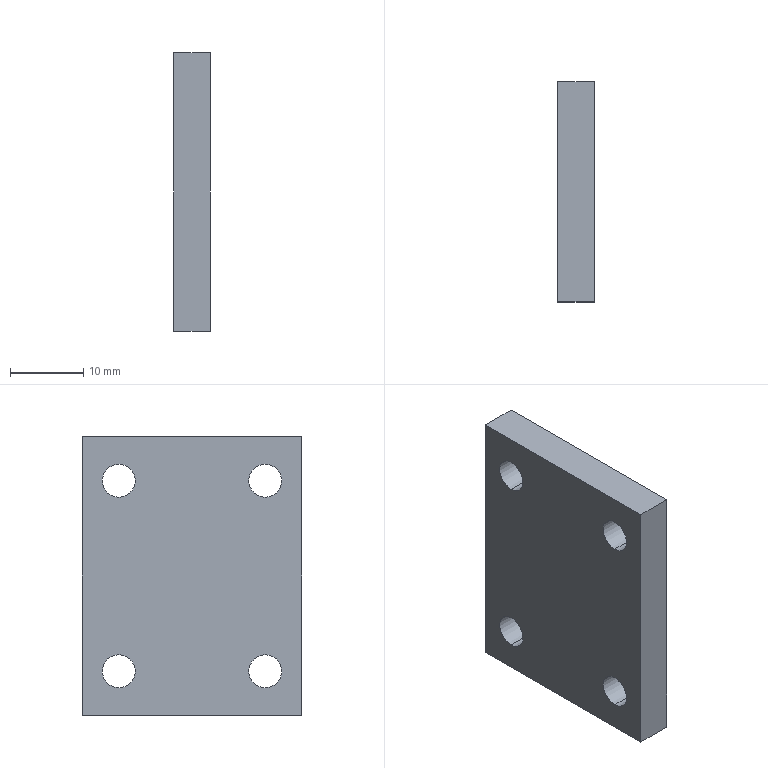Component | SolidWorks | DC-024-30-1 | 1 solid | 14 faces | box 5 x 30 x 38 mm | volume 5382 mm3 | cylinder 8 | plane 6 | commonest cylinder face diameters 4.5 x8
build123d program:
from build123d import *

# Parameters (mm, degrees)
SKETCH1_W                  = 38
SKETCH1_H                  = 30
BOSS_EXTRUDE1_DEPTH        = 2.5
F_4_5_4_5_DIAMETER_HOLE1_D = 4.5


with BuildPart() as part:
    # Sketch1 → Boss-Extrude1 (new, symmetric)
    with BuildSketch(Plane.XY):
        Rectangle(SKETCH1_W, SKETCH1_H)
    extrude(amount=BOSS_EXTRUDE1_DEPTH, both=True)

    # 4.5 _4.5_ Diameter Hole1 (through all)
    with Locations(Plane.XY.offset(2.5)):
        with Locations((-13, 10), (-13, -10), (13, -10), (13, 10)):
            Hole(F_4_5_4_5_DIAMETER_HOLE1_D / 2)


solid = part.part

# Placed as in the assembly
solid = solid.moved(Location((-65.833, 220.806, 37), (0, 90, 0)))
STEP:
#1=COLOUR_RGB('',0.7922,0.8196,0.9333);
#2=FILL_AREA_STYLE_COLOUR('',#1);
#3=FILL_AREA_STYLE('',(#2));
#4=SURFACE_STYLE_FILL_AREA(#3);
#5=SURFACE_SIDE_STYLE('',(#4));
#6=SURFACE_STYLE_USAGE(.BOTH.,#5);
#7=PRESENTATION_STYLE_ASSIGNMENT((#6));
#8=CARTESIAN_POINT('',(-2.69,9.087,2.057));
#9=VERTEX_POINT('',#8);
#10=CARTESIAN_POINT('',(-2.69,9.087,1.88));
#11=VERTEX_POINT('',#10);
#12=CARTESIAN_POINT('',(-2.69,9.087,1.969));
#13=DIRECTION('',(1.,-0.,0.));
#14=DIRECTION('',(0.,0.,-1.));
#15=AXIS2_PLACEMENT_3D('',#12,#13,#14);
#16=CIRCLE('',#15,0.08858);
#17=EDGE_CURVE('',#9,#11,#16,.T.);
#18=ORIENTED_EDGE('',*,*,#17,.F.);
#19=CARTESIAN_POINT('',(-2.493,9.087,2.057));
#20=VERTEX_POINT('',#19);
#21=CARTESIAN_POINT('',(-2.493,9.087,2.057));
#22=DIRECTION('',(1.,-0.,0.));
#23=VECTOR('',#22,39.37);
#24=LINE('',#21,#23);
#25=EDGE_CURVE('',#9,#20,#24,.T.);
#26=ORIENTED_EDGE('',*,*,#25,.T.);
#27=CARTESIAN_POINT('',(-2.493,9.087,1.88));
#28=VERTEX_POINT('',#27);
#29=CARTESIAN_POINT('',(-2.493,9.087,1.969));
#30=DIRECTION('',(1.,-0.,0.));
#31=DIRECTION('',(0.,0.,-1.));
#32=AXIS2_PLACEMENT_3D('',#29,#30,#31);
#33=CIRCLE('',#32,0.08858);
#34=EDGE_CURVE('',#20,#28,#33,.T.);
#35=ORIENTED_EDGE('',*,*,#34,.T.);
#36=CARTESIAN_POINT('',(-2.493,9.087,1.88));
#37=DIRECTION('',(1.,-0.,0.));
#38=VECTOR('',#37,39.37);
#39=LINE('',#36,#38);
#40=EDGE_CURVE('',#11,#28,#39,.T.);
#41=ORIENTED_EDGE('',*,*,#40,.F.);
#42=EDGE_LOOP('',(#18,#26,#35,#41));
#43=FACE_OUTER_BOUND('',#42,.T.);
#44=CARTESIAN_POINT('',(-2.493,9.087,1.969));
#45=DIRECTION('',(1.,-0.,0.));
#46=DIRECTION('',(0.,0.,-1.));
#47=AXIS2_PLACEMENT_3D('',#44,#45,#46);
#48=CYLINDRICAL_SURFACE('',#47,0.08858);
#49=ADVANCED_FACE('',(#43),#48,.F.);
#50=CARTESIAN_POINT('',(-2.69,8.299,2.057));
#51=VERTEX_POINT('',#50);
#52=CARTESIAN_POINT('',(-2.69,8.299,1.88));
#53=VERTEX_POINT('',#52);
#54=CARTESIAN_POINT('',(-2.69,8.299,1.969));
#55=DIRECTION('',(1.,-0.,0.));
#56=DIRECTION('',(0.,0.,-1.));
#57=AXIS2_PLACEMENT_3D('',#54,#55,#56);
#58=CIRCLE('',#57,0.08858);
#59=EDGE_CURVE('',#51,#53,#58,.T.);
#60=ORIENTED_EDGE('',*,*,#59,.F.);
#61=CARTESIAN_POINT('',(-2.493,8.299,2.057));
#62=VERTEX_POINT('',#61);
#63=CARTESIAN_POINT('',(-2.493,8.299,2.057));
#64=DIRECTION('',(1.,-0.,0.));
#65=VECTOR('',#64,39.37);
#66=LINE('',#63,#65);
#67=EDGE_CURVE('',#51,#62,#66,.T.);
#68=ORIENTED_EDGE('',*,*,#67,.T.);
#69=CARTESIAN_POINT('',(-2.493,8.299,1.88));
#70=VERTEX_POINT('',#69);
#71=CARTESIAN_POINT('',(-2.493,8.299,1.969));
#72=DIRECTION('',(1.,-0.,0.));
#73=DIRECTION('',(0.,0.,-1.));
#74=AXIS2_PLACEMENT_3D('',#71,#72,#73);
#75=CIRCLE('',#74,0.08858);
#76=EDGE_CURVE('',#62,#70,#75,.T.);
#77=ORIENTED_EDGE('',*,*,#76,.T.);
#78=CARTESIAN_POINT('',(-2.493,8.299,1.88));
#79=DIRECTION('',(1.,-0.,0.));
#80=VECTOR('',#79,39.37);
#81=LINE('',#78,#80);
#82=EDGE_CURVE('',#53,#70,#81,.T.);
#83=ORIENTED_EDGE('',*,*,#82,.F.);
#84=EDGE_LOOP('',(#60,#68,#77,#83));
#85=FACE_OUTER_BOUND('',#84,.T.);
#86=CARTESIAN_POINT('',(-2.493,8.299,1.969));
#87=DIRECTION('',(1.,-0.,0.));
#88=DIRECTION('',(0.,0.,-1.));
#89=AXIS2_PLACEMENT_3D('',#86,#87,#88);
#90=CYLINDRICAL_SURFACE('',#89,0.08858);
#91=ADVANCED_FACE('',(#85),#90,.F.);
#92=CARTESIAN_POINT('',(-2.69,8.299,1.033));
#93=VERTEX_POINT('',#92);
#94=CARTESIAN_POINT('',(-2.69,8.299,0.8563));
#95=VERTEX_POINT('',#94);
#96=CARTESIAN_POINT('',(-2.69,8.299,0.9449));
#97=DIRECTION('',(1.,-0.,0.));
#98=DIRECTION('',(0.,0.,-1.));
#99=AXIS2_PLACEMENT_3D('',#96,#97,#98);
#100=CIRCLE('',#99,0.08858);
#101=EDGE_CURVE('',#93,#95,#100,.T.);
#102=ORIENTED_EDGE('',*,*,#101,.F.);
#103=CARTESIAN_POINT('',(-2.493,8.299,1.033));
#104=VERTEX_POINT('',#103);
#105=CARTESIAN_POINT('',(-2.493,8.299,1.033));
#106=DIRECTION('',(1.,-0.,0.));
#107=VECTOR('',#106,39.37);
#108=LINE('',#105,#107);
#109=EDGE_CURVE('',#93,#104,#108,.T.);
#110=ORIENTED_EDGE('',*,*,#109,.T.);
#111=CARTESIAN_POINT('',(-2.493,8.299,0.8563));
#112=VERTEX_POINT('',#111);
#113=CARTESIAN_POINT('',(-2.493,8.299,0.9449));
#114=DIRECTION('',(1.,-0.,0.));
#115=DIRECTION('',(0.,0.,-1.));
#116=AXIS2_PLACEMENT_3D('',#113,#114,#115);
#117=CIRCLE('',#116,0.08858);
#118=EDGE_CURVE('',#104,#112,#117,.T.);
#119=ORIENTED_EDGE('',*,*,#118,.T.);
#120=CARTESIAN_POINT('',(-2.493,8.299,0.8563));
#121=DIRECTION('',(1.,-0.,0.));
#122=VECTOR('',#121,39.37);
#123=LINE('',#120,#122);
#124=EDGE_CURVE('',#95,#112,#123,.T.);
#125=ORIENTED_EDGE('',*,*,#124,.F.);
#126=EDGE_LOOP('',(#102,#110,#119,#125));
#127=FACE_OUTER_BOUND('',#126,.T.);
#128=CARTESIAN_POINT('',(-2.493,8.299,0.9449));
#129=DIRECTION('',(1.,-0.,0.));
#130=DIRECTION('',(0.,0.,-1.));
#131=AXIS2_PLACEMENT_3D('',#128,#129,#130);
#132=CYLINDRICAL_SURFACE('',#131,0.08858);
#133=ADVANCED_FACE('',(#127),#132,.F.);
#134=CARTESIAN_POINT('',(-2.69,9.087,1.033));
#135=VERTEX_POINT('',#134);
#136=CARTESIAN_POINT('',(-2.69,9.087,0.8563));
#137=VERTEX_POINT('',#136);
#138=CARTESIAN_POINT('',(-2.69,9.087,0.9449));
#139=DIRECTION('',(1.,-0.,0.));
#140=DIRECTION('',(0.,0.,-1.));
#141=AXIS2_PLACEMENT_3D('',#138,#139,#140);
#142=CIRCLE('',#141,0.08858);
#143=EDGE_CURVE('',#135,#137,#142,.T.);
#144=ORIENTED_EDGE('',*,*,#143,.F.);
#145=CARTESIAN_POINT('',(-2.493,9.087,1.033));
#146=VERTEX_POINT('',#145);
#147=CARTESIAN_POINT('',(-2.493,9.087,1.033));
#148=DIRECTION('',(1.,-0.,0.));
#149=VECTOR('',#148,39.37);
#150=LINE('',#147,#149);
#151=EDGE_CURVE('',#135,#146,#150,.T.);
#152=ORIENTED_EDGE('',*,*,#151,.T.);
#153=CARTESIAN_POINT('',(-2.493,9.087,0.8563));
#154=VERTEX_POINT('',#153);
#155=CARTESIAN_POINT('',(-2.493,9.087,0.9449));
#156=DIRECTION('',(1.,-0.,0.));
#157=DIRECTION('',(0.,0.,-1.));
#158=AXIS2_PLACEMENT_3D('',#155,#156,#157);
#159=CIRCLE('',#158,0.08858);
#160=EDGE_CURVE('',#146,#154,#159,.T.);
#161=ORIENTED_EDGE('',*,*,#160,.T.);
#162=CARTESIAN_POINT('',(-2.493,9.087,0.8563));
#163=DIRECTION('',(1.,-0.,0.));
#164=VECTOR('',#163,39.37);
#165=LINE('',#162,#164);
#166=EDGE_CURVE('',#137,#154,#165,.T.);
#167=ORIENTED_EDGE('',*,*,#166,.F.);
#168=EDGE_LOOP('',(#144,#152,#161,#167));
#169=FACE_OUTER_BOUND('',#168,.T.);
#170=CARTESIAN_POINT('',(-2.493,9.087,0.9449));
#171=DIRECTION('',(1.,-0.,0.));
#172=DIRECTION('',(0.,0.,-1.));
#173=AXIS2_PLACEMENT_3D('',#170,#171,#172);
#174=CYLINDRICAL_SURFACE('',#173,0.08858);
#175=ADVANCED_FACE('',(#169),#174,.F.);
#176=CARTESIAN_POINT('',(-2.69,9.284,2.205));
#177=VERTEX_POINT('',#176);
#178=CARTESIAN_POINT('',(-2.69,8.103,2.205));
#179=VERTEX_POINT('',#178);
#180=CARTESIAN_POINT('',(-2.69,8.103,2.205));
#181=DIRECTION('',(-0.,-1.,-0.));
#182=VECTOR('',#181,39.37);
#183=LINE('',#180,#182);
#184=EDGE_CURVE('',#177,#179,#183,.T.);
#185=ORIENTED_EDGE('',*,*,#184,.T.);
#186=CARTESIAN_POINT('',(-2.493,8.103,2.205));
#187=VERTEX_POINT('',#186);
#188=CARTESIAN_POINT('',(-2.493,8.103,2.205));
#189=DIRECTION('',(-1.,0.,-0.));
#190=VECTOR('',#189,39.37);
#191=LINE('',#188,#190);
#192=EDGE_CURVE('',#187,#179,#191,.T.);
#193=ORIENTED_EDGE('',*,*,#192,.F.);
#194=CARTESIAN_POINT('',(-2.493,9.284,2.205));
#195=VERTEX_POINT('',#194);
#196=CARTESIAN_POINT('',(-2.493,8.103,2.205));
#197=DIRECTION('',(-0.,-1.,-0.));
#198=VECTOR('',#197,39.37);
#199=LINE('',#196,#198);
#200=EDGE_CURVE('',#195,#187,#199,.T.);
#201=ORIENTED_EDGE('',*,*,#200,.F.);
#202=CARTESIAN_POINT('',(-2.493,9.284,2.205));
#203=DIRECTION('',(-1.,0.,-0.));
#204=VECTOR('',#203,39.37);
#205=LINE('',#202,#204);
#206=EDGE_CURVE('',#195,#177,#205,.T.);
#207=ORIENTED_EDGE('',*,*,#206,.T.);
#208=EDGE_LOOP('',(#185,#193,#201,#207));
#209=FACE_OUTER_BOUND('',#208,.T.);
#210=CARTESIAN_POINT('',(-2.493,8.103,2.205));
#211=DIRECTION('',(0.,0.,-1.));
#212=DIRECTION('',(-1.,0.,-0.));
#213=AXIS2_PLACEMENT_3D('',#210,#211,#212);
#214=PLANE('',#213);
#215=ADVANCED_FACE('',(#209),#214,.F.);
#216=CARTESIAN_POINT('',(-2.69,8.103,0.7087));
#217=VERTEX_POINT('',#216);
#218=CARTESIAN_POINT('',(-2.69,8.103,0.7087));
#219=DIRECTION('',(0.,0.,-1.));
#220=VECTOR('',#219,39.37);
#221=LINE('',#218,#220);
#222=EDGE_CURVE('',#179,#217,#221,.T.);
#223=ORIENTED_EDGE('',*,*,#222,.T.);
#224=CARTESIAN_POINT('',(-2.493,8.103,0.7087));
#225=VERTEX_POINT('',#224);
#226=CARTESIAN_POINT('',(-2.493,8.103,0.7087));
#227=DIRECTION('',(-1.,0.,-0.));
#228=VECTOR('',#227,39.37);
#229=LINE('',#226,#228);
#230=EDGE_CURVE('',#225,#217,#229,.T.);
#231=ORIENTED_EDGE('',*,*,#230,.F.);
#232=CARTESIAN_POINT('',(-2.493,8.103,0.7087));
#233=DIRECTION('',(0.,0.,-1.));
#234=VECTOR('',#233,39.37);
#235=LINE('',#232,#234);
#236=EDGE_CURVE('',#187,#225,#235,.T.);
#237=ORIENTED_EDGE('',*,*,#236,.F.);
#238=ORIENTED_EDGE('',*,*,#192,.T.);
#239=EDGE_LOOP('',(#223,#231,#237,#238));
#240=FACE_OUTER_BOUND('',#239,.T.);
#241=CARTESIAN_POINT('',(-2.493,8.103,0.7087));
#242=DIRECTION('',(0.,1.,0.));
#243=DIRECTION('',(-0.,-0.,1.));
#244=AXIS2_PLACEMENT_3D('',#241,#242,#243);
#245=PLANE('',#244);
#246=ADVANCED_FACE('',(#240),#245,.F.);
#247=CARTESIAN_POINT('',(-2.69,9.284,0.7087));
#248=VERTEX_POINT('',#247);
#249=CARTESIAN_POINT('',(-2.69,8.103,0.7087));
#250=DIRECTION('',(0.,1.,0.));
#251=VECTOR('',#250,39.37);
#252=LINE('',#249,#251);
#253=EDGE_CURVE('',#217,#248,#252,.T.);
#254=ORIENTED_EDGE('',*,*,#253,.T.);
#255=CARTESIAN_POINT('',(-2.493,9.284,0.7087));
#256=VERTEX_POINT('',#255);
#257=CARTESIAN_POINT('',(-2.493,9.284,0.7087));
#258=DIRECTION('',(-1.,0.,-0.));
#259=VECTOR('',#258,39.37);
#260=LINE('',#257,#259);
#261=EDGE_CURVE('',#256,#248,#260,.T.);
#262=ORIENTED_EDGE('',*,*,#261,.F.);
#263=CARTESIAN_POINT('',(-2.493,8.103,0.7087));
#264=DIRECTION('',(0.,1.,0.));
#265=VECTOR('',#264,39.37);
#266=LINE('',#263,#265);
#267=EDGE_CURVE('',#225,#256,#266,.T.);
#268=ORIENTED_EDGE('',*,*,#267,.F.);
#269=ORIENTED_EDGE('',*,*,#230,.T.);
#270=EDGE_LOOP('',(#254,#262,#268,#269));
#271=FACE_OUTER_BOUND('',#270,.T.);
#272=CARTESIAN_POINT('',(-2.493,8.103,0.7087));
#273=DIRECTION('',(-0.,-0.,1.));
#274=DIRECTION('',(1.,-0.,0.));
#275=AXIS2_PLACEMENT_3D('',#272,#273,#274);
#276=PLANE('',#275);
#277=ADVANCED_FACE('',(#271),#276,.F.);
#278=CARTESIAN_POINT('',(-2.69,9.284,0.7087));
#279=DIRECTION('',(-0.,-0.,1.));
#280=VECTOR('',#279,39.37);
#281=LINE('',#278,#280);
#282=EDGE_CURVE('',#248,#177,#281,.T.);
#283=ORIENTED_EDGE('',*,*,#282,.T.);
#284=ORIENTED_EDGE('',*,*,#206,.F.);
#285=CARTESIAN_POINT('',(-2.493,9.284,0.7087));
#286=DIRECTION('',(-0.,-0.,1.));
#287=VECTOR('',#286,39.37);
#288=LINE('',#285,#287);
#289=EDGE_CURVE('',#256,#195,#288,.T.);
#290=ORIENTED_EDGE('',*,*,#289,.F.);
#291=ORIENTED_EDGE('',*,*,#261,.T.);
#292=EDGE_LOOP('',(#283,#284,#290,#291));
#293=FACE_OUTER_BOUND('',#292,.T.);
#294=CARTESIAN_POINT('',(-2.493,9.284,0.7087));
#295=DIRECTION('',(-0.,-1.,-0.));
#296=DIRECTION('',(0.,0.,-1.));
#297=AXIS2_PLACEMENT_3D('',#294,#295,#296);
#298=PLANE('',#297);
#299=ADVANCED_FACE('',(#293),#298,.F.);
#300=CARTESIAN_POINT('',(-2.493,9.087,1.969));
#301=DIRECTION('',(1.,-0.,0.));
#302=DIRECTION('',(0.,0.,-1.));
#303=AXIS2_PLACEMENT_3D('',#300,#301,#302);
#304=CIRCLE('',#303,0.08858);
#305=EDGE_CURVE('',#28,#20,#304,.T.);
#306=ORIENTED_EDGE('',*,*,#305,.F.);
#307=ORIENTED_EDGE('',*,*,#34,.F.);
#308=EDGE_LOOP('',(#306,#307));
#309=FACE_BOUND('',#308,.T.);
#310=CARTESIAN_POINT('',(-2.493,8.299,1.969));
#311=DIRECTION('',(1.,-0.,0.));
#312=DIRECTION('',(0.,0.,-1.));
#313=AXIS2_PLACEMENT_3D('',#310,#311,#312);
#314=CIRCLE('',#313,0.08858);
#315=EDGE_CURVE('',#70,#62,#314,.T.);
#316=ORIENTED_EDGE('',*,*,#315,.F.);
#317=ORIENTED_EDGE('',*,*,#76,.F.);
#318=EDGE_LOOP('',(#316,#317));
#319=FACE_BOUND('',#318,.T.);
#320=CARTESIAN_POINT('',(-2.493,8.299,0.9449));
#321=DIRECTION('',(1.,-0.,0.));
#322=DIRECTION('',(0.,0.,-1.));
#323=AXIS2_PLACEMENT_3D('',#320,#321,#322);
#324=CIRCLE('',#323,0.08858);
#325=EDGE_CURVE('',#112,#104,#324,.T.);
#326=ORIENTED_EDGE('',*,*,#325,.F.);
#327=ORIENTED_EDGE('',*,*,#118,.F.);
#328=EDGE_LOOP('',(#326,#327));
#329=FACE_BOUND('',#328,.T.);
#330=CARTESIAN_POINT('',(-2.493,9.087,0.9449));
#331=DIRECTION('',(1.,-0.,0.));
#332=DIRECTION('',(0.,0.,-1.));
#333=AXIS2_PLACEMENT_3D('',#330,#331,#332);
#334=CIRCLE('',#333,0.08858);
#335=EDGE_CURVE('',#154,#146,#334,.T.);
#336=ORIENTED_EDGE('',*,*,#335,.F.);
#337=ORIENTED_EDGE('',*,*,#160,.F.);
#338=EDGE_LOOP('',(#336,#337));
#339=FACE_BOUND('',#338,.T.);
#340=ORIENTED_EDGE('',*,*,#200,.T.);
#341=ORIENTED_EDGE('',*,*,#236,.T.);
#342=ORIENTED_EDGE('',*,*,#267,.T.);
#343=ORIENTED_EDGE('',*,*,#289,.T.);
#344=EDGE_LOOP('',(#340,#341,#342,#343));
#345=FACE_OUTER_BOUND('',#344,.T.);
#346=CARTESIAN_POINT('',(-2.493,8.693,1.457));
#347=DIRECTION('',(1.,-0.,0.));
#348=DIRECTION('',(0.,0.,-1.));
#349=AXIS2_PLACEMENT_3D('',#346,#347,#348);
#350=PLANE('',#349);
#351=ADVANCED_FACE('',(#309,#319,#329,#339,#345),#350,.T.);
#352=CARTESIAN_POINT('',(-2.69,9.087,1.969));
#353=DIRECTION('',(1.,-0.,0.));
#354=DIRECTION('',(0.,0.,-1.));
#355=AXIS2_PLACEMENT_3D('',#352,#353,#354);
#356=CIRCLE('',#355,0.08858);
#357=EDGE_CURVE('',#11,#9,#356,.T.);
#358=ORIENTED_EDGE('',*,*,#357,.T.);
#359=ORIENTED_EDGE('',*,*,#17,.T.);
#360=EDGE_LOOP('',(#358,#359));
#361=FACE_BOUND('',#360,.T.);
#362=CARTESIAN_POINT('',(-2.69,8.299,1.969));
#363=DIRECTION('',(1.,-0.,0.));
#364=DIRECTION('',(0.,0.,-1.));
#365=AXIS2_PLACEMENT_3D('',#362,#363,#364);
#366=CIRCLE('',#365,0.08858);
#367=EDGE_CURVE('',#53,#51,#366,.T.);
#368=ORIENTED_EDGE('',*,*,#367,.T.);
#369=ORIENTED_EDGE('',*,*,#59,.T.);
#370=EDGE_LOOP('',(#368,#369));
#371=FACE_BOUND('',#370,.T.);
#372=CARTESIAN_POINT('',(-2.69,8.299,0.9449));
#373=DIRECTION('',(1.,-0.,0.));
#374=DIRECTION('',(0.,0.,-1.));
#375=AXIS2_PLACEMENT_3D('',#372,#373,#374);
#376=CIRCLE('',#375,0.08858);
#377=EDGE_CURVE('',#95,#93,#376,.T.);
#378=ORIENTED_EDGE('',*,*,#377,.T.);
#379=ORIENTED_EDGE('',*,*,#101,.T.);
#380=EDGE_LOOP('',(#378,#379));
#381=FACE_BOUND('',#380,.T.);
#382=CARTESIAN_POINT('',(-2.69,9.087,0.9449));
#383=DIRECTION('',(1.,-0.,0.));
#384=DIRECTION('',(0.,0.,-1.));
#385=AXIS2_PLACEMENT_3D('',#382,#383,#384);
#386=CIRCLE('',#385,0.08858);
#387=EDGE_CURVE('',#137,#135,#386,.T.);
#388=ORIENTED_EDGE('',*,*,#387,.T.);
#389=ORIENTED_EDGE('',*,*,#143,.T.);
#390=EDGE_LOOP('',(#388,#389));
#391=FACE_BOUND('',#390,.T.);
#392=ORIENTED_EDGE('',*,*,#184,.F.);
#393=ORIENTED_EDGE('',*,*,#282,.F.);
#394=ORIENTED_EDGE('',*,*,#253,.F.);
#395=ORIENTED_EDGE('',*,*,#222,.F.);
#396=EDGE_LOOP('',(#392,#393,#394,#395));
#397=FACE_OUTER_BOUND('',#396,.T.);
#398=CARTESIAN_POINT('',(-2.69,8.693,1.457));
#399=DIRECTION('',(1.,-0.,0.));
#400=DIRECTION('',(0.,0.,-1.));
#401=AXIS2_PLACEMENT_3D('',#398,#399,#400);
#402=PLANE('',#401);
#403=ADVANCED_FACE('',(#361,#371,#381,#391,#397),#402,.F.);
#404=ORIENTED_EDGE('',*,*,#151,.F.);
#405=ORIENTED_EDGE('',*,*,#387,.F.);
#406=ORIENTED_EDGE('',*,*,#166,.T.);
#407=ORIENTED_EDGE('',*,*,#335,.T.);
#408=EDGE_LOOP('',(#404,#405,#406,#407));
#409=FACE_OUTER_BOUND('',#408,.T.);
#410=CARTESIAN_POINT('',(-2.493,9.087,0.9449));
#411=DIRECTION('',(1.,-0.,0.));
#412=DIRECTION('',(0.,0.,-1.));
#413=AXIS2_PLACEMENT_3D('',#410,#411,#412);
#414=CYLINDRICAL_SURFACE('',#413,0.08858);
#415=ADVANCED_FACE('',(#409),#414,.F.);
#416=ORIENTED_EDGE('',*,*,#109,.F.);
#417=ORIENTED_EDGE('',*,*,#377,.F.);
#418=ORIENTED_EDGE('',*,*,#124,.T.);
#419=ORIENTED_EDGE('',*,*,#325,.T.);
#420=EDGE_LOOP('',(#416,#417,#418,#419));
#421=FACE_OUTER_BOUND('',#420,.T.);
#422=CARTESIAN_POINT('',(-2.493,8.299,0.9449));
#423=DIRECTION('',(1.,-0.,0.));
#424=DIRECTION('',(0.,0.,-1.));
#425=AXIS2_PLACEMENT_3D('',#422,#423,#424);
#426=CYLINDRICAL_SURFACE('',#425,0.08858);
#427=ADVANCED_FACE('',(#421),#426,.F.);
#428=ORIENTED_EDGE('',*,*,#67,.F.);
#429=ORIENTED_EDGE('',*,*,#367,.F.);
#430=ORIENTED_EDGE('',*,*,#82,.T.);
#431=ORIENTED_EDGE('',*,*,#315,.T.);
#432=EDGE_LOOP('',(#428,#429,#430,#431));
#433=FACE_OUTER_BOUND('',#432,.T.);
#434=CARTESIAN_POINT('',(-2.493,8.299,1.969));
#435=DIRECTION('',(1.,-0.,0.));
#436=DIRECTION('',(0.,0.,-1.));
#437=AXIS2_PLACEMENT_3D('',#434,#435,#436);
#438=CYLINDRICAL_SURFACE('',#437,0.08858);
#439=ADVANCED_FACE('',(#433),#438,.F.);
#440=ORIENTED_EDGE('',*,*,#25,.F.);
#441=ORIENTED_EDGE('',*,*,#357,.F.);
#442=ORIENTED_EDGE('',*,*,#40,.T.);
#443=ORIENTED_EDGE('',*,*,#305,.T.);
#444=EDGE_LOOP('',(#440,#441,#442,#443));
#445=FACE_OUTER_BOUND('',#444,.T.);
#446=CARTESIAN_POINT('',(-2.493,9.087,1.969));
#447=DIRECTION('',(1.,-0.,0.));
#448=DIRECTION('',(0.,0.,-1.));
#449=AXIS2_PLACEMENT_3D('',#446,#447,#448);
#450=CYLINDRICAL_SURFACE('',#449,0.08858);
#451=ADVANCED_FACE('',(#445),#450,.F.);
#452=CLOSED_SHELL('',(#49,#91,#133,#175,#215,#246,#277,#299,#351,#403,#415,#427,#439,#451));
#453=MANIFOLD_SOLID_BREP('',#452);
#454=STYLED_ITEM('',(#7),#453);
#455=(LENGTH_UNIT()NAMED_UNIT(*)SI_UNIT($,.METRE.));
#456=LENGTH_MEASURE_WITH_UNIT(LENGTH_MEASURE(0.0254),#455);
#457=DIMENSIONAL_EXPONENTS(1.,0.,0.,0.,0.,0.,0.);
#458=(CONVERSION_BASED_UNIT('',#456)LENGTH_UNIT()NAMED_UNIT(#457));
#459=UNCERTAINTY_MEASURE_WITH_UNIT(LENGTH_MEASURE(0.00001),#458,'','');
#460=(NAMED_UNIT(*)PLANE_ANGLE_UNIT()SI_UNIT($,.RADIAN.));
#461=(NAMED_UNIT(*)SI_UNIT($,.STERADIAN.)SOLID_ANGLE_UNIT());
#462=(GEOMETRIC_REPRESENTATION_CONTEXT(3)GLOBAL_UNCERTAINTY_ASSIGNED_CONTEXT((#459))GLOBAL_UNIT_ASSIGNED_CONTEXT((#458,#460,#461))REPRESENTATION_CONTEXT('',''));
#463=MECHANICAL_DESIGN_GEOMETRIC_PRESENTATION_REPRESENTATION('',(#454),#462);
#464=PRESENTATION_LAYER_ASSIGNMENT('','',(#454));
#465=CARTESIAN_POINT('',(0.,0.,0.));
#466=DIRECTION('',(0.,0.,1.));
#467=DIRECTION('',(1.,0.,0.));
#468=AXIS2_PLACEMENT_3D('',#465,#466,#467);
#469=(LENGTH_UNIT()NAMED_UNIT(*)SI_UNIT($,.METRE.));
#470=LENGTH_MEASURE_WITH_UNIT(LENGTH_MEASURE(0.0254),#469);
#471=DIMENSIONAL_EXPONENTS(1.,0.,0.,0.,0.,0.,0.);
#472=(CONVERSION_BASED_UNIT('',#470)LENGTH_UNIT()NAMED_UNIT(#471));
#473=UNCERTAINTY_MEASURE_WITH_UNIT(LENGTH_MEASURE(0.00001),#472,'','');
#474=(NAMED_UNIT(*)PLANE_ANGLE_UNIT()SI_UNIT($,.RADIAN.));
#475=(NAMED_UNIT(*)SI_UNIT($,.STERADIAN.)SOLID_ANGLE_UNIT());
#476=(GEOMETRIC_REPRESENTATION_CONTEXT(3)GLOBAL_UNCERTAINTY_ASSIGNED_CONTEXT((#473))GLOBAL_UNIT_ASSIGNED_CONTEXT((#472,#474,#475))REPRESENTATION_CONTEXT('',''));
#477=ADVANCED_BREP_SHAPE_REPRESENTATION('',(#453,#468),#476);